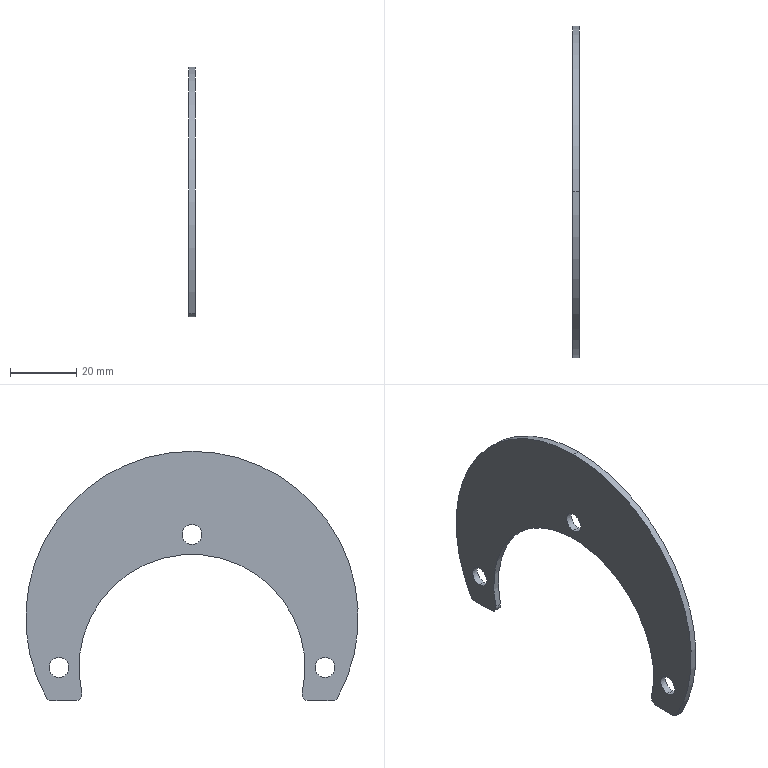Component | SolidWorks | ChainPartFrontCover-1 | 1 solid | 17 faces | box 2 x 100 x 75 mm | volume 7489 mm3 | cylinder 13 | plane 4 | commonest cylinder face diameters 6 x6 4 x4 100 x2 68 x1
build123d program:
from build123d import *

# Parameters (mm, degrees)
BOSS_EXTRUDE1_DEPTH = 1
SKETCH4_R           = 34
CUT_EXTRUDE2_DEPTH  = 71.739
SKETCH3_R           = 3
CUT_EXTRUDE1_DEPTH  = 71.739
FILLET1_R           = 2


with BuildPart() as part:
    # Sketch2 → Boss-Extrude1 (new, symmetric)
    with BuildSketch(Plane.XY):
        with BuildLine():
            Line((25, 43.301), (25, -43.301))
            ThreePointArc((25, -43.301), (-50, 0), (25, 43.301))
        make_face()
    extrude(amount=BOSS_EXTRUDE1_DEPTH, both=True)

    # Sketch4 → Cut-Extrude2 (cut, through all)
    with BuildSketch(Plane.XY.offset(1)):
        with Locations((15, 0)):
            Circle(SKETCH4_R)
    extrude(amount=-CUT_EXTRUDE2_DEPTH, mode=Mode.SUBTRACT)

    # Sketch3 → Cut-Extrude1 (cut, through all)
    with BuildSketch(Plane.XY.offset(1)):
        with Locations((15, 40)):
            Circle(SKETCH3_R)
        with Locations((-25, 0)):
            Circle(SKETCH3_R)
        with Locations((15, -40)):
            Circle(SKETCH3_R)
    extrude(amount=-CUT_EXTRUDE1_DEPTH, mode=Mode.SUBTRACT)

    # Fillet1
    fillet1_edges = [part.edges().sort_by_distance(p)[0] for p in [
        (25, -32.496, 0),
        (25, 32.496, 0),
        (25, 43.301, 0),
        (25, -43.301, 0),
    ]]
    fillet(fillet1_edges, radius=FILLET1_R)


solid = part.part

# Placed as in the assembly
solid = solid.moved(Location((79.237, -2.563, -20.304), (0, 90, 0)))